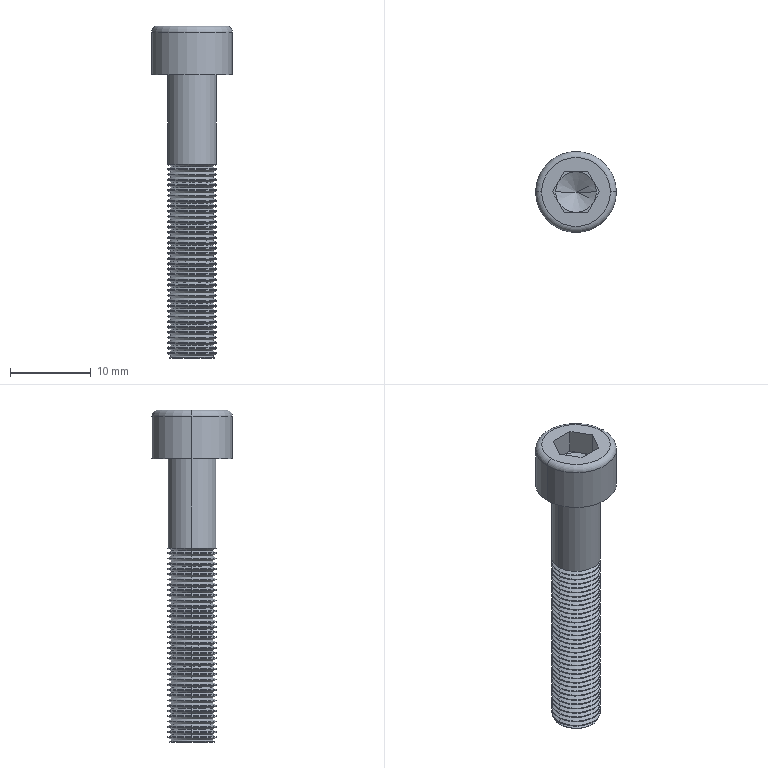Component | SolidWorks | RetractableStop-LongSide-1_HexagonSocketHeadCapScrew-M6X35-0510-1 | 1 solid | 245 faces | box 10 x 10 x 41 mm | volume 1299 mm3 | cone 152 | cylinder 76 | plane 15 | torus 2 | commonest cylinder face diameters 6 x74 10 x2
build123d program:
from build123d import *

# Parameters (mm, degrees)
SKETCH1_R           = 5
BASEHEAD_DEPTH      = 6
SKETCH2_R           = 3
BASEBODY_DEPTH      = 35
HEXAGONSOCKET_DEPTH = 3
TOPFILLET_R         = 0.75
CHAMFER1_SIZE       = 0.25
LPATTERN10_COUNT    = 37
LPATTERN10_PITCH    = 0.6498


with BuildPart() as part:
    # Sketch1 → BaseHead (new body)
    with BuildSketch(Plane(origin=(0, 0, 0), x_dir=(0, 0, -1), z_dir=(1, 0, 0))):
        Circle(SKETCH1_R)
    extrude(amount=BASEHEAD_DEPTH)

    # Sketch2 → BaseBody (add)
    with BuildSketch(Plane(origin=(6, 0, 0), x_dir=(0, 0, -1), z_dir=(1, 0, 0))):
        Circle(SKETCH2_R)
    extrude(amount=BASEBODY_DEPTH)

    # Sketch3 → HexagonSocket (cut)
    with BuildSketch(Plane(origin=(0, 0, 0), x_dir=(0, 0, -1), z_dir=(1, 0, 0))):
        Polygon((2.887, 0), (1.443, 2.5), (-1.443, 2.5), (-2.887, 0), (-1.443, -2.5), (1.443, -2.5), align=None)
    extrude(amount=HEXAGONSOCKET_DEPTH, mode=Mode.SUBTRACT)

    # Sketch4 → Cut-Revolve1 (revolve, cut)
    with BuildSketch(Plane(origin=(-4.196, 0.75, 0), x_dir=(-1, 0, 0), z_dir=(0, 0, 1)), mode=Mode.PRIVATE) as cut_revolve1_sk:
        Polygon((-7.196, 3.25), (-8.64, 0.75), (-7.196, 0.75), align=None)
    revolve(cut_revolve1_sk.sketch.rotate(Axis((0.839, 0, 0), (-1, 0, 0)), 90), axis=Axis((0.839, 0, 0), (-1, 0, 0)), mode=Mode.SUBTRACT)

    # TopFillet
    topfillet_edges = [part.edges().sort_by_distance(p)[0] for p in [
        (0, 0, 5),
    ]]
    fillet(topfillet_edges, radius=TOPFILLET_R)

    # Chamfer1
    chamfer1_edges = [part.edges().sort_by_distance(p)[0] for p in [
        (41, 0, 3),
    ]]
    chamfer(chamfer1_edges, length=CHAMFER1_SIZE)

    # Sketch5 → Cut-Revolve10 (revolve, cut)
    with BuildSketch(Plane.XY, mode=Mode.PRIVATE) as cut_revolve10_sk:
        Polygon((40.75, 2.531), (41.021, 3), (41.021, 3.542), (40.479, 3.542), (40.479, 3), align=None)
    cut_revolve10 = revolve(cut_revolve10_sk.sketch.rotate(Axis((0, 0, 0), (1, 0, 0)), 90), axis=Axis((0, 0, 0), (1, 0, 0)), mode=Mode.SUBTRACT)

    # LPattern10: Cut-Revolve10 ×37
    with Locations(*[(-i * LPATTERN10_PITCH, 0, 0) for i in range(1, LPATTERN10_COUNT)]):
        add(cut_revolve10, mode=Mode.SUBTRACT)


solid = part.part

# Placed as in the assembly
solid = solid.moved(Location((-1369.513, 43.736, 3578.5), (0, 90, 0)))